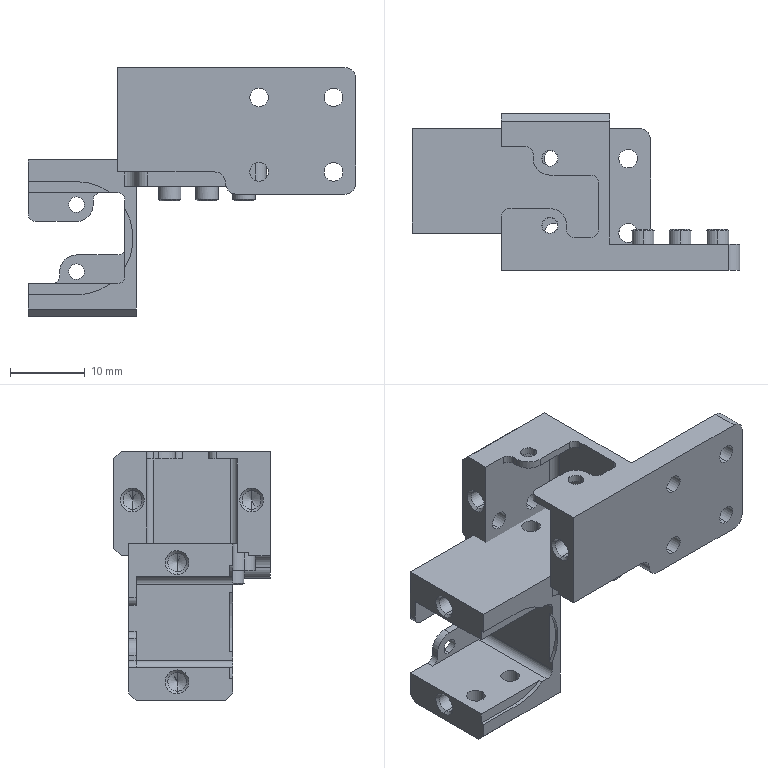CAM job | Mastercam | mm | 40 operations | part box 44 x 21 x 33.4
1. 3D High Speed (Dynamic OptiRough) | 2 - 10C
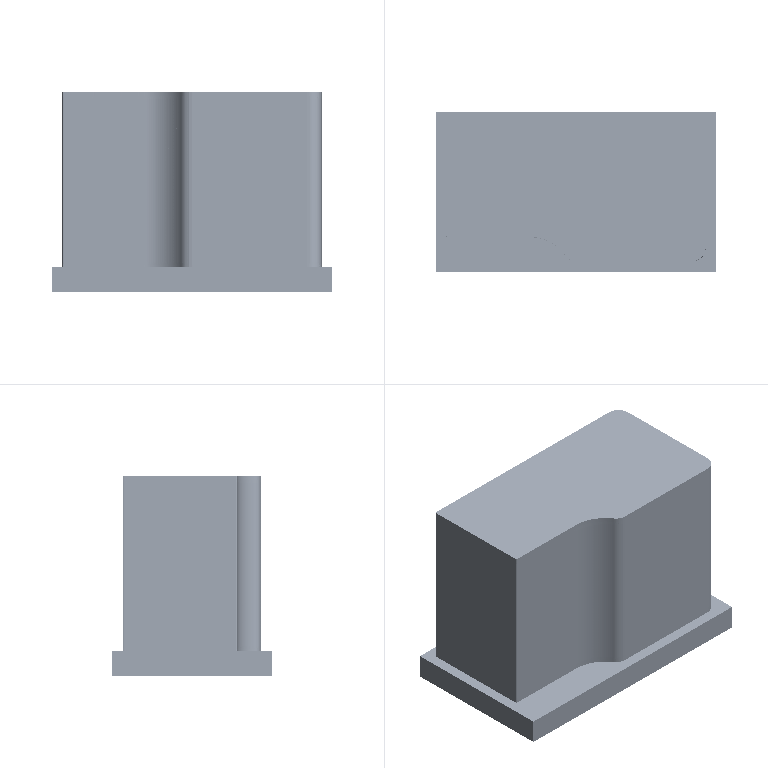2. Drill/Counterbore | 6 - 6 倒角刀
3. Peck Drill | 8 - 2.5 钻头
4. Facing | 3 - 10J
5. Contour (2D) | 3 - 10J
6. Contour (Remachining) | 27 - 3 平铣刀
7. Model Chamfer | 6 - 6 倒角刀
8. Drill/Counterbore | 6 - 6 倒角刀
9. Peck Drill | 8 - 2.5 钻头
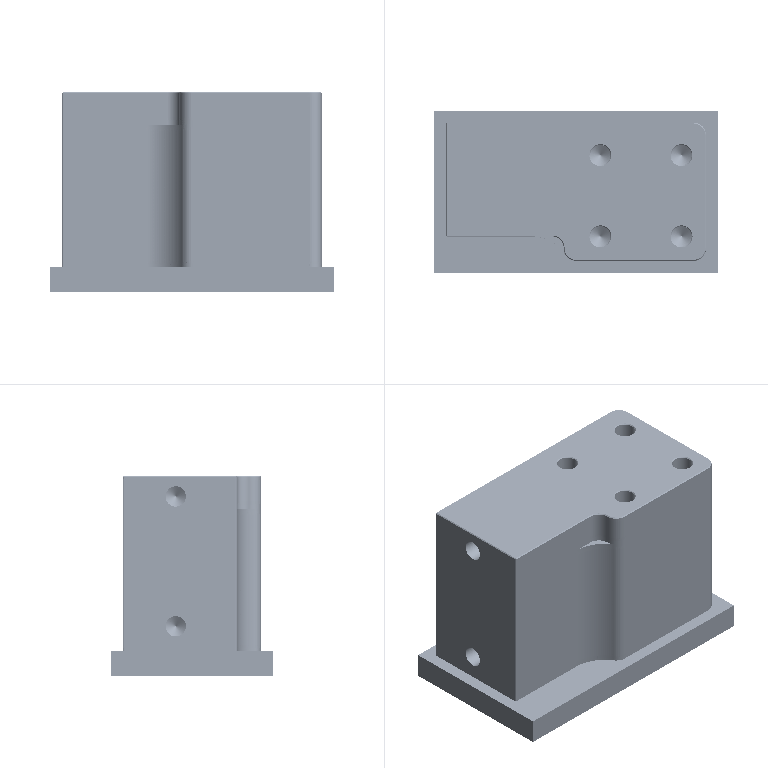10. Chamfer Drill | 6 - 6 倒角刀
11. Drill/Counterbore | 6 - 6 倒角刀
12. Peck Drill | 29 - 2.1 钻头
13. 2D High Speed (2D Area Mill) | 4 - 4C
14. Contour (2D) | 5 - 4J
15. Contour (Remachining) | 13 - 2J
16. Contour (2D chamfer) | 6 - 6 倒角刀
17. Chamfer Drill | 6 - 6 倒角刀
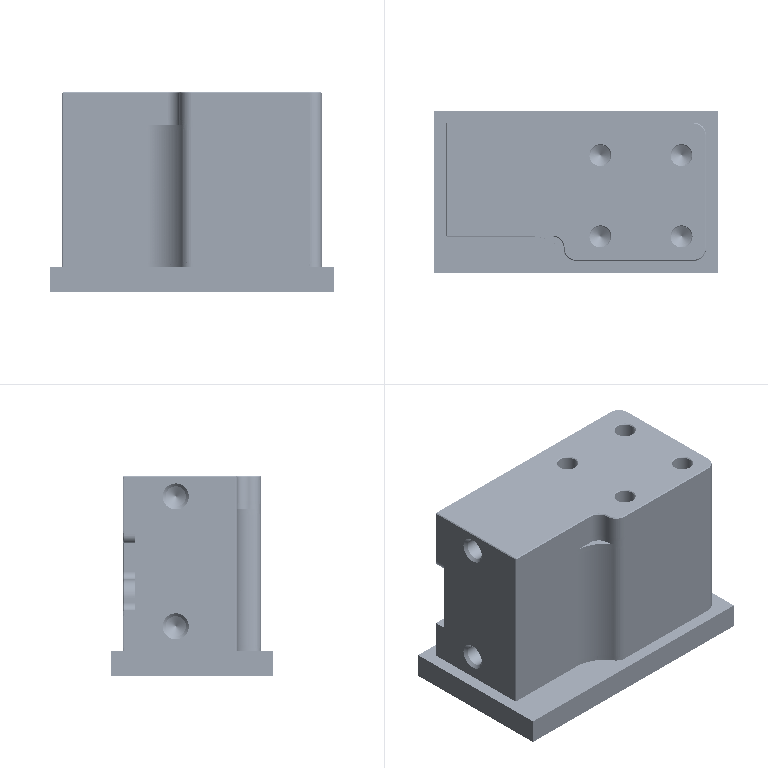18. Facing | 2 - 10C
19. 3D High Speed (Area rest roughing) | 4 - 4C
20. Facing | 3 - 10J
21. Contour (2D) | 5 - 4J
22. 3D High Speed (Horizontal) | 5 - 4J
23. 3D High Speed (Area rest roughing) | 12 - 2C
24. Triangular mesh Triangular mesh | 13 - 2J
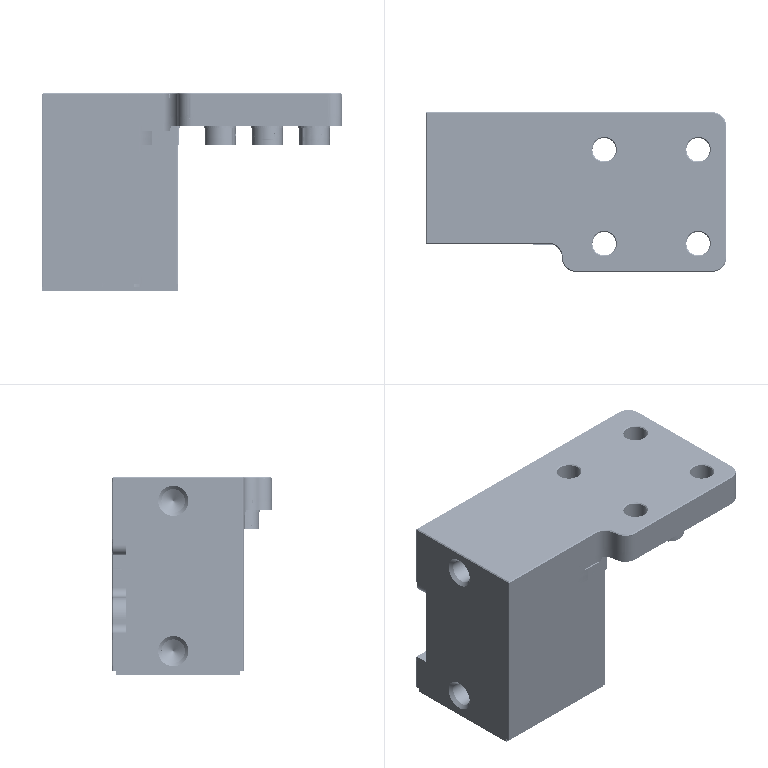25. Contour (2D) | 13 - 2J
26. Contour (2D) | 13 - 2J
27. Drill/Counterbore | 6 - 6 倒角刀
28. Peck Drill | 8 - 2.5 钻头
29. Chamfer Drill | 6 - 6 倒角刀
30. Contour (2D chamfer) | 6 - 6 倒角刀
31. Contour (2D chamfer) | 6 - 6 倒角刀
32. Contour (2D chamfer) | 11 - 4 倒角刀
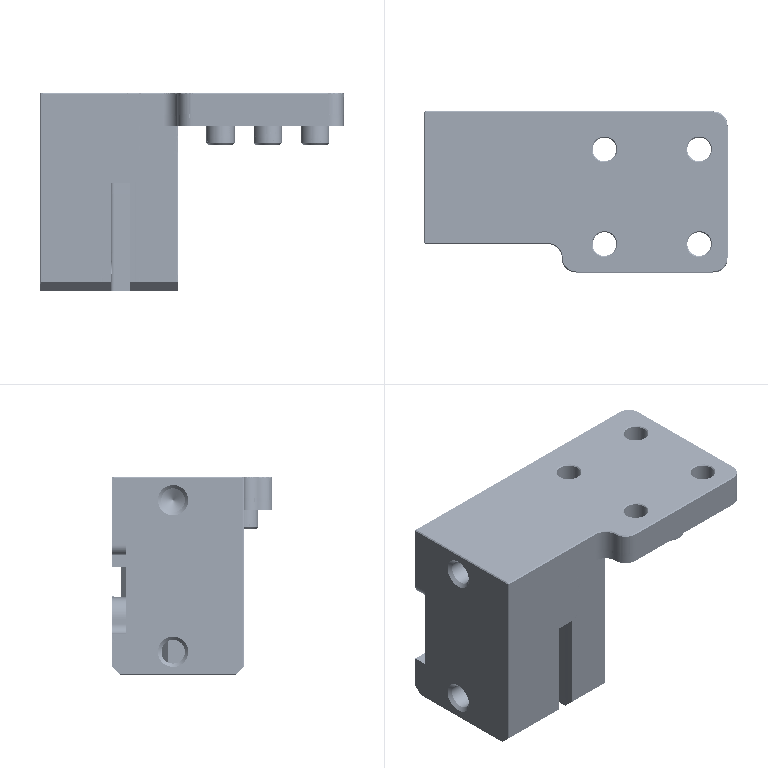33. Chamfer Drill | 11 - 4 倒角刀
34. Model Chamfer | 11 - 4 倒角刀
35. 3D High Speed (Area rest roughing) | 4 - 4C
36. Triangular mesh Triangular mesh | 5 - 4J
37. Contour (2D) | 5 - 4J
38. Contour (2D) | 5 - 4J
39. Contour (Remachining) | 13 - 2J
40. Model Chamfer | 11 - 4 倒角刀